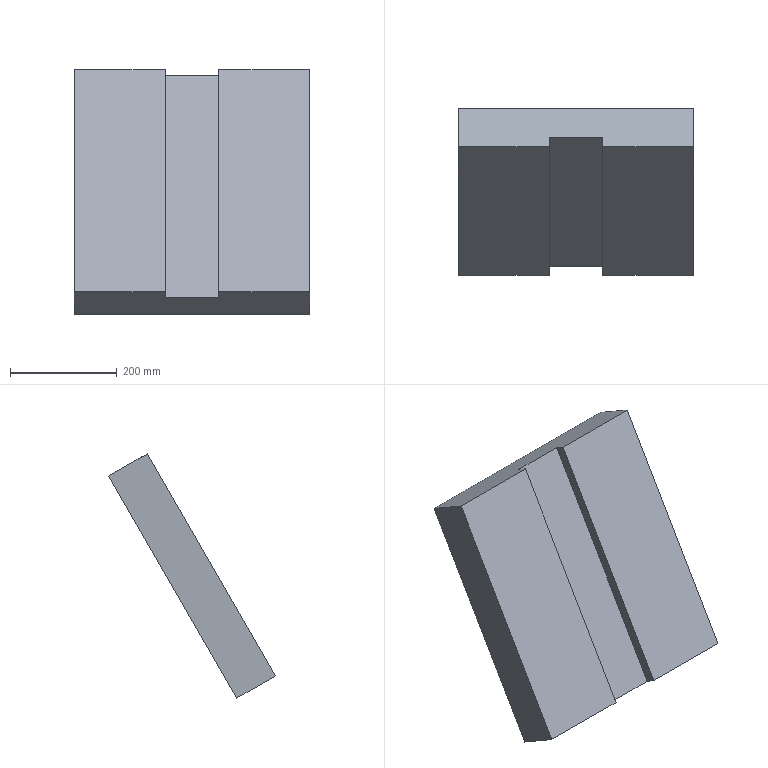Component | NX | SIM15_Z2_SCHLITTEN | 1 solid | 10 faces | volume 16569600 mm3 | plane 10